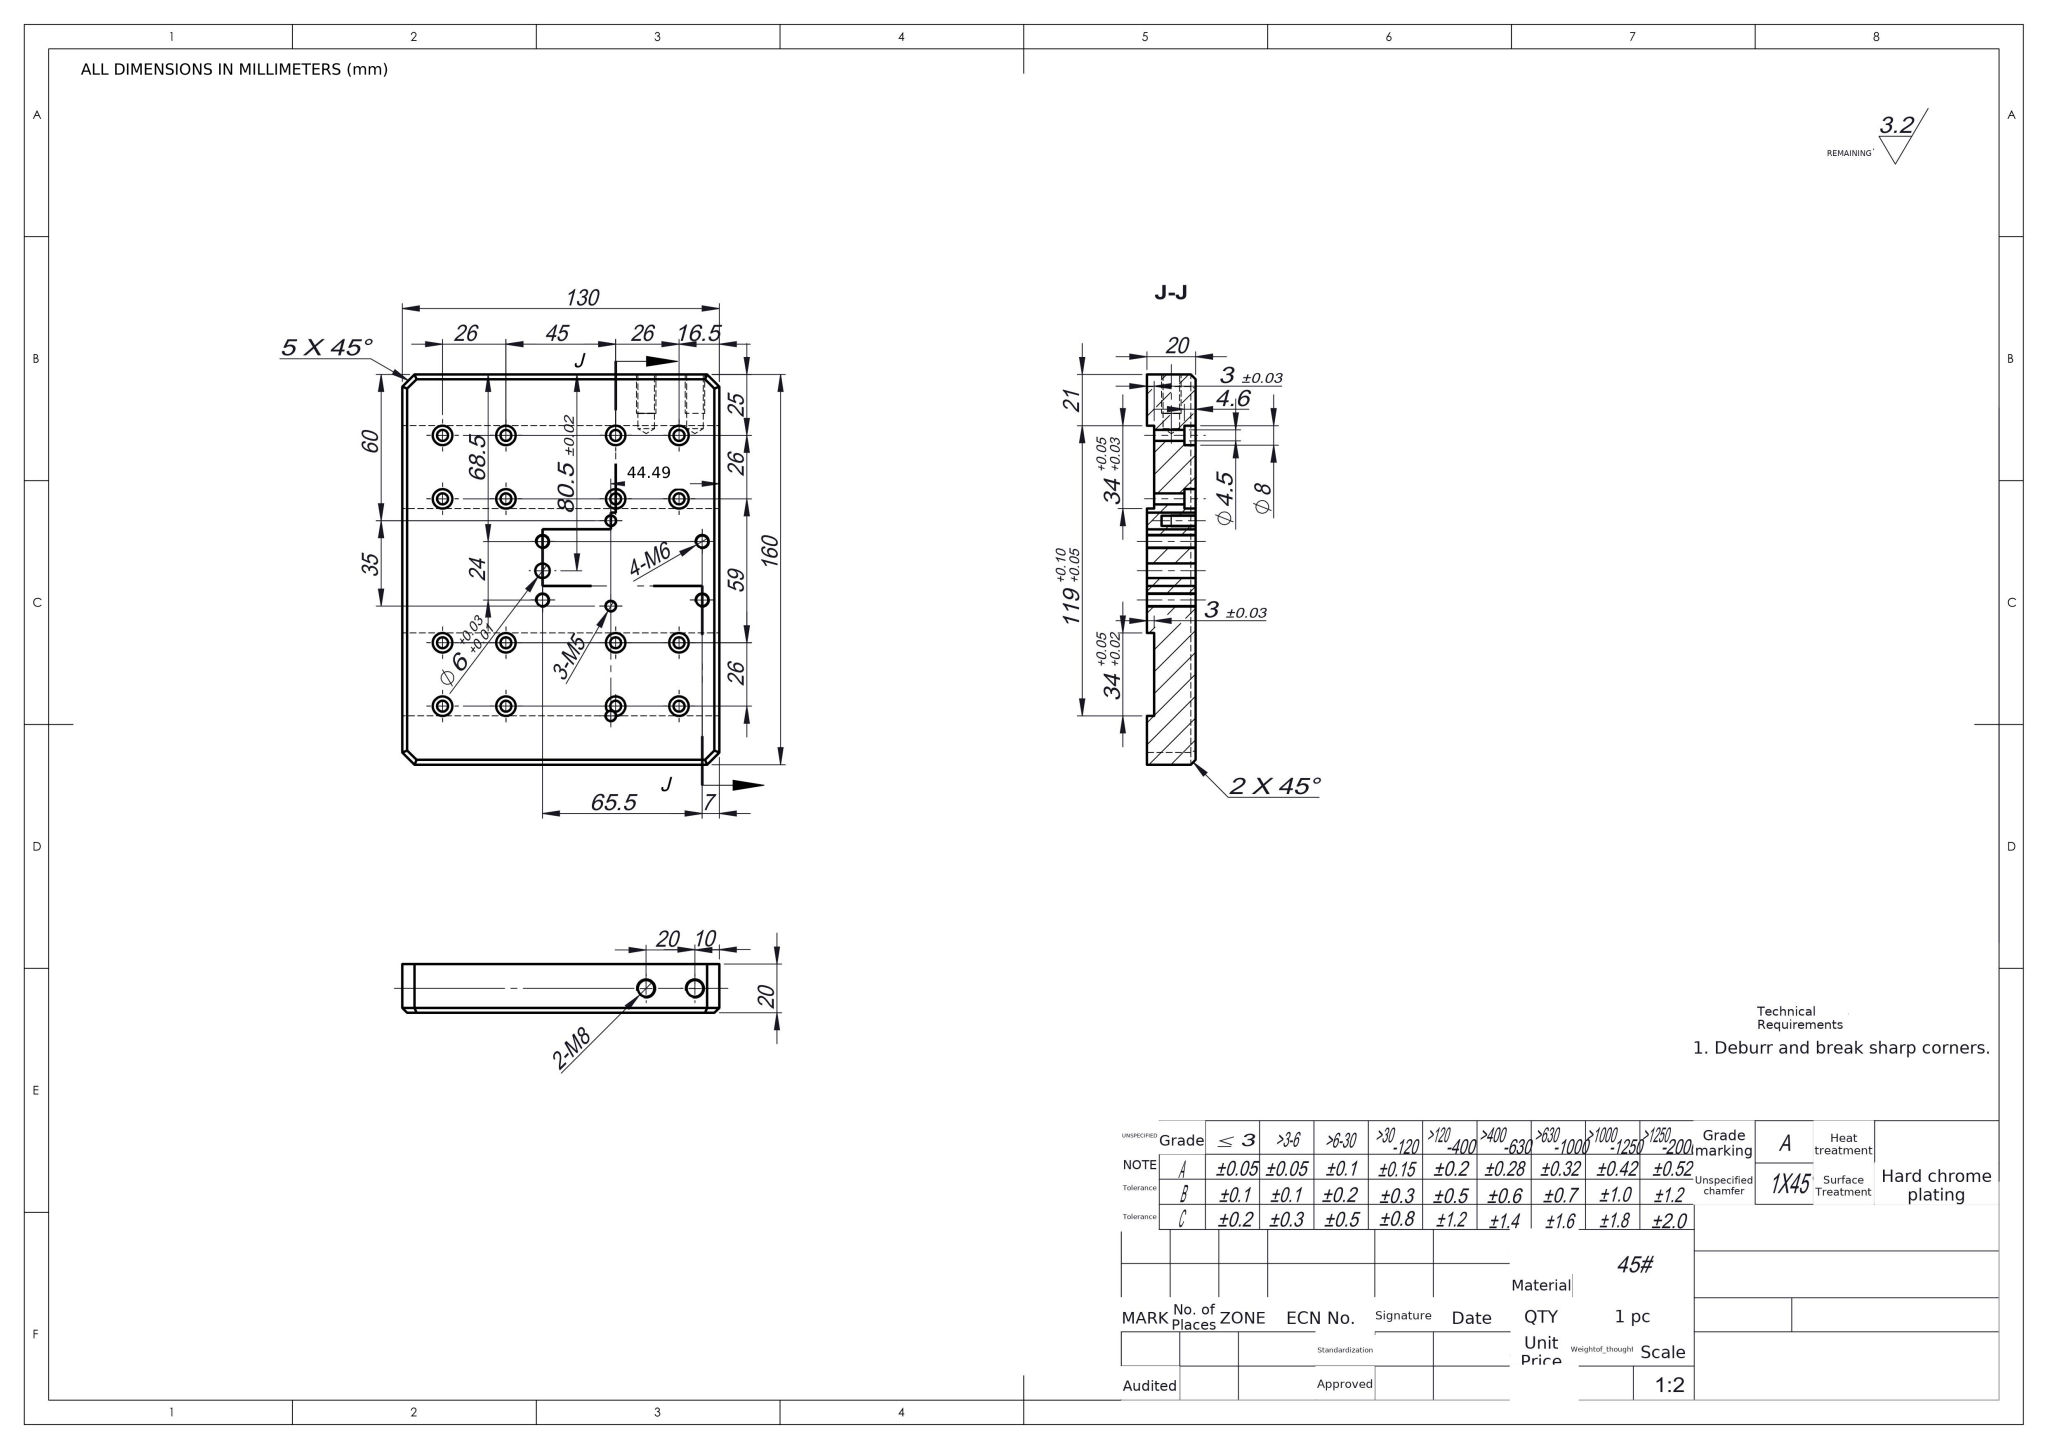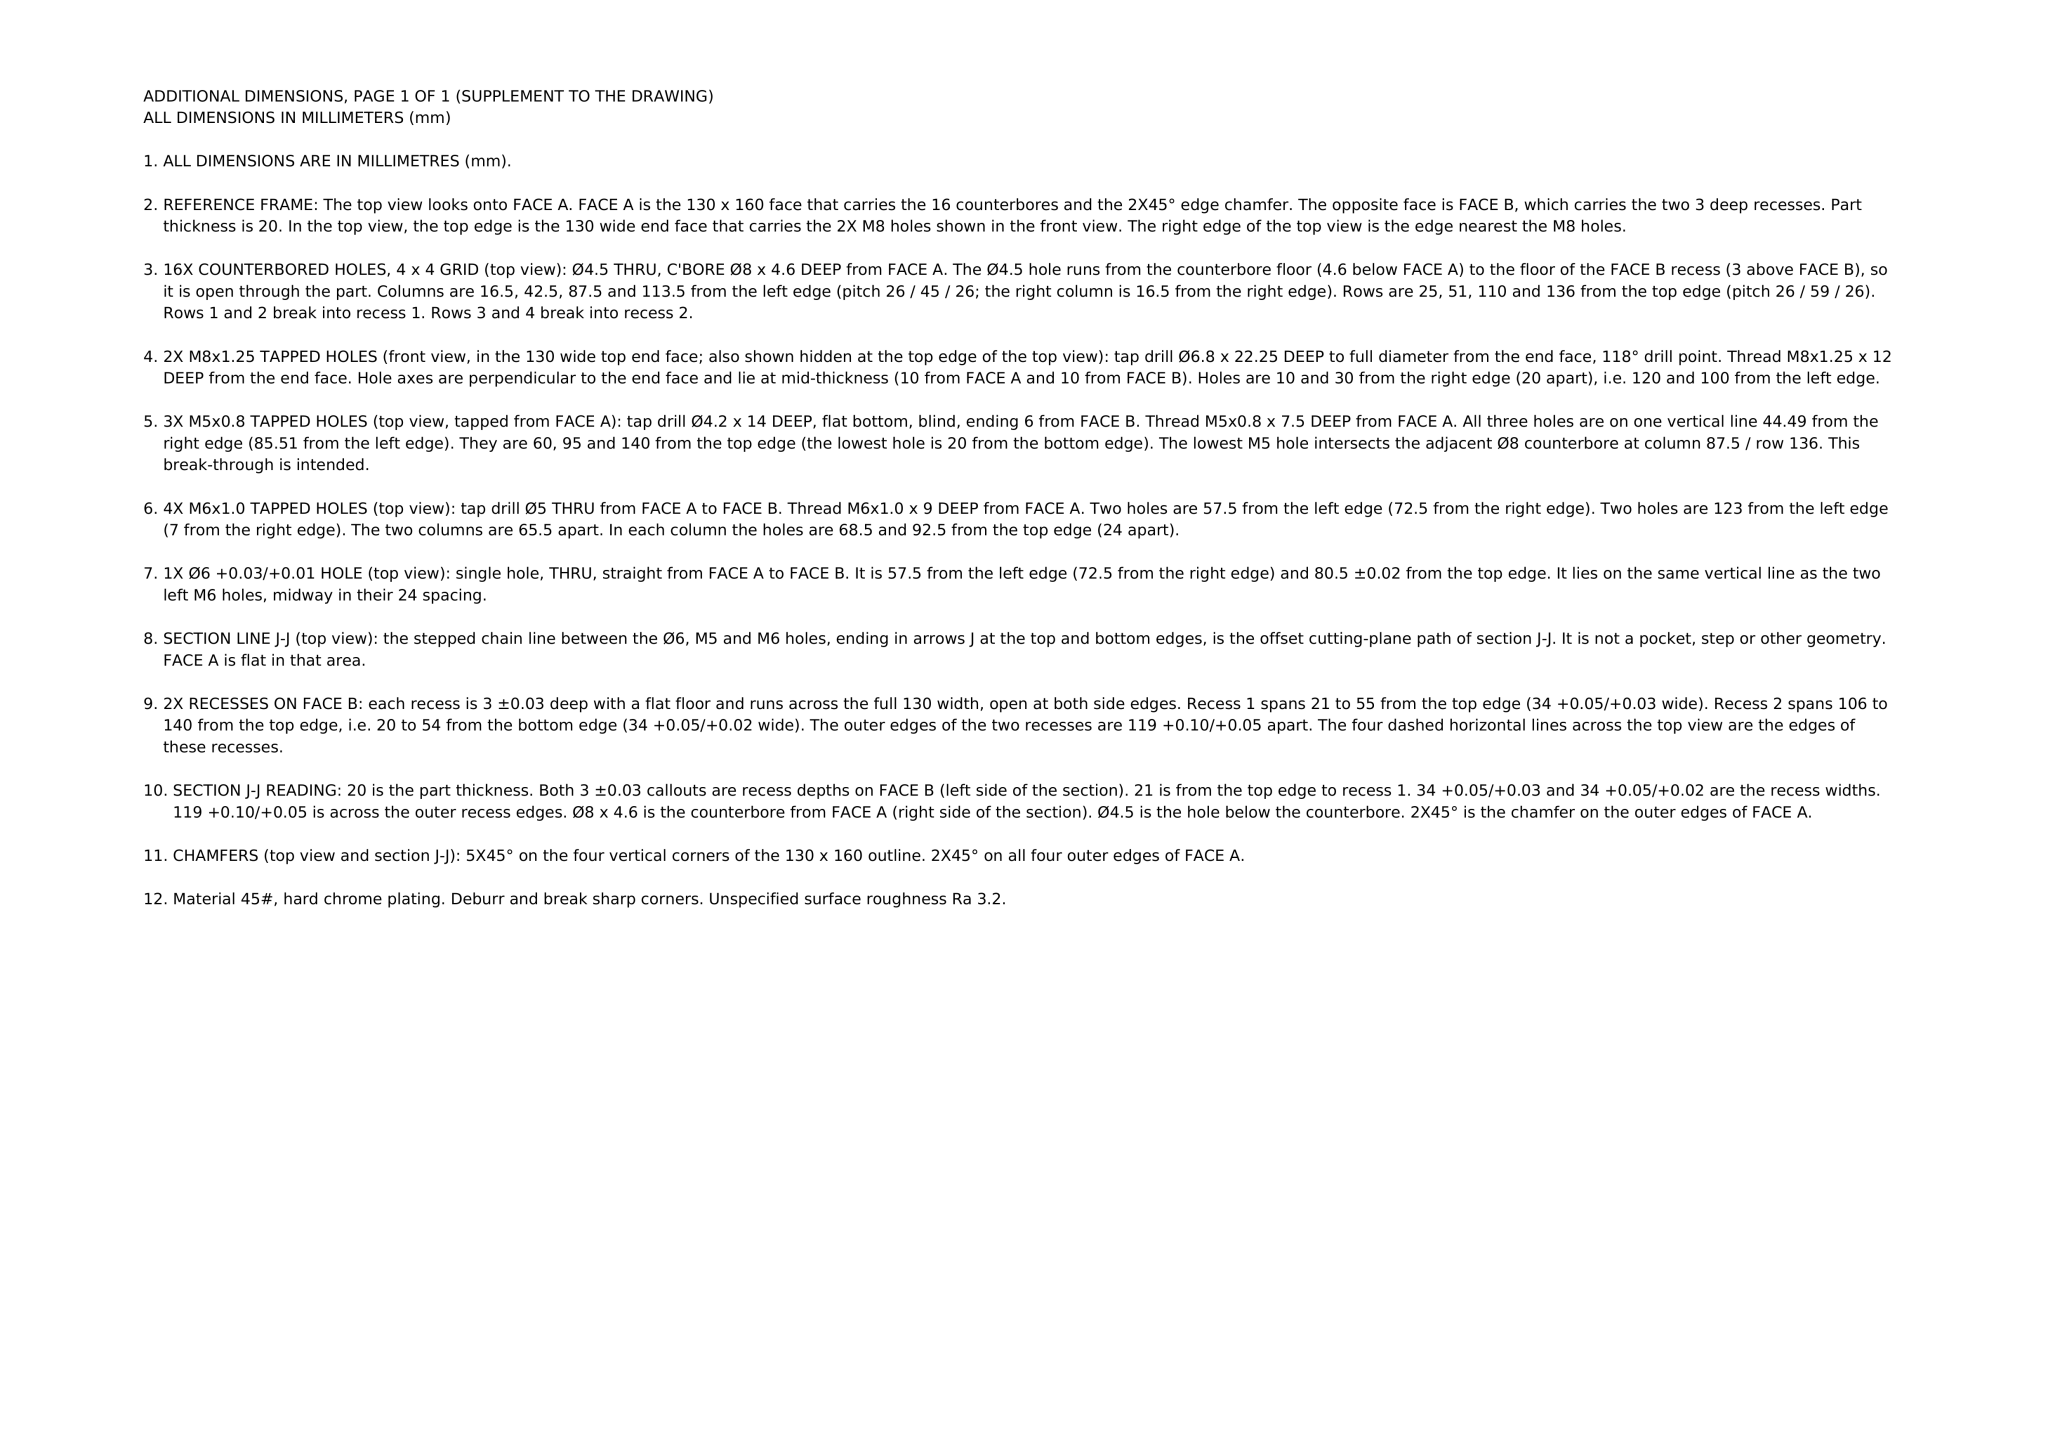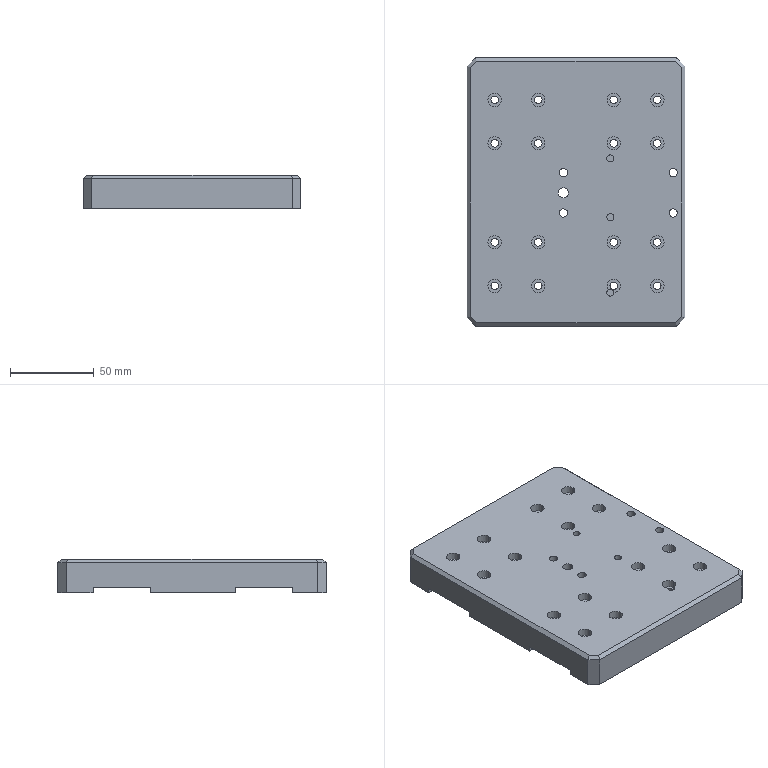Part | NX | mm | 1 solid | 134 faces | box 130 x 160 x 20 mm | volume 376133 mm3 | cylinder 85 | plane 45 | cone 4 | commonest cylinder face diameters 8 x33 4.5 x32 5 x8 4.2 x6 6.8 x4 6 x2